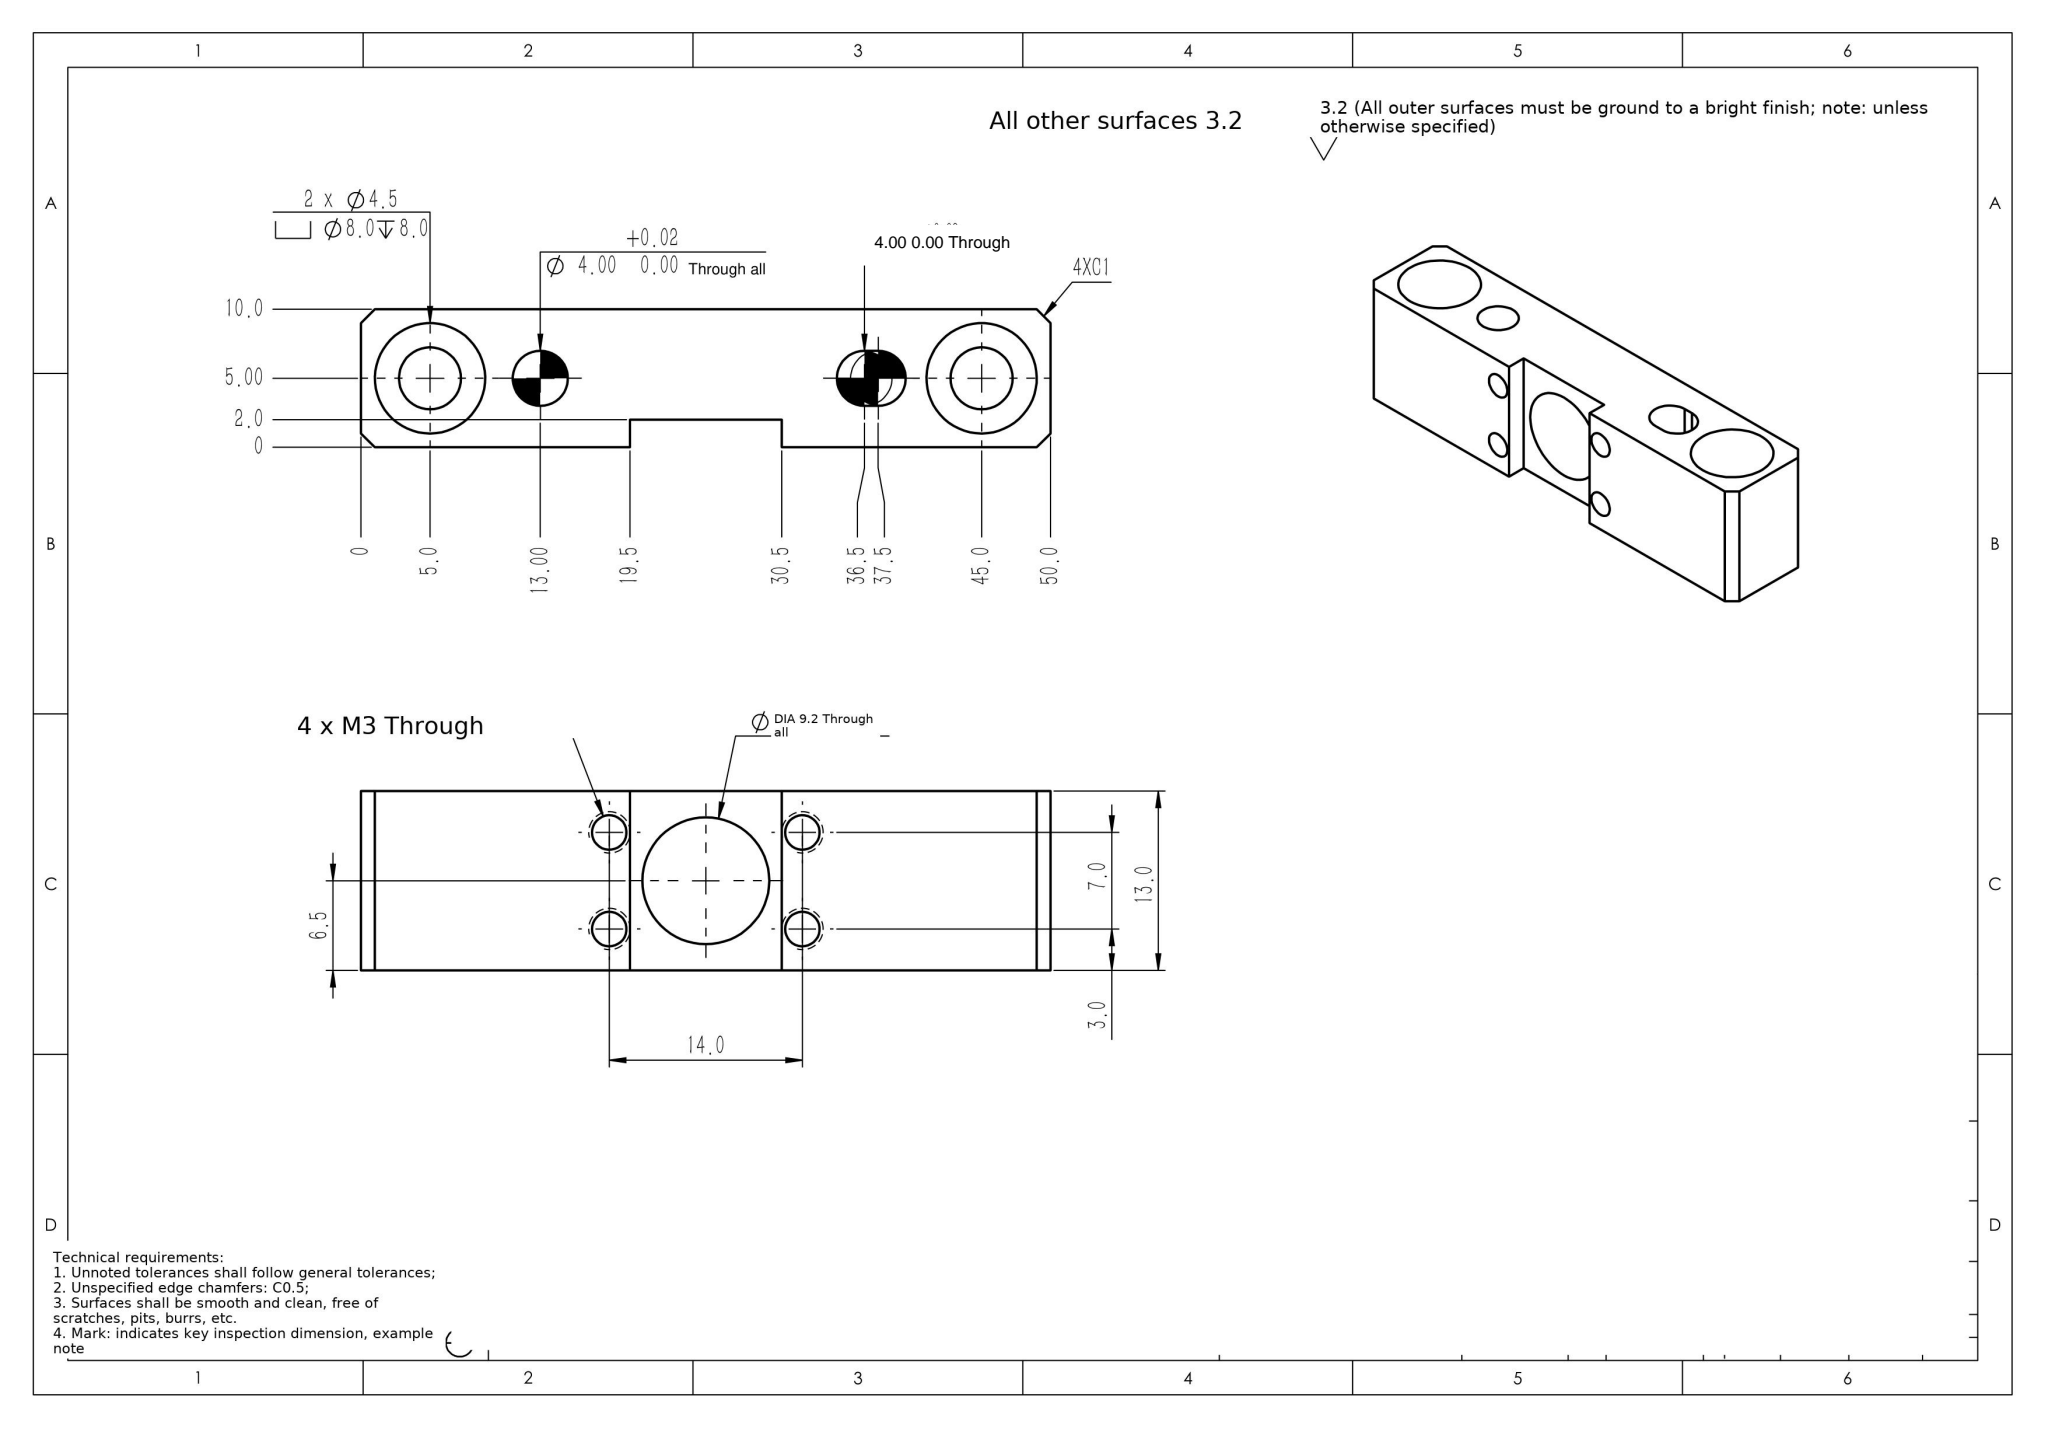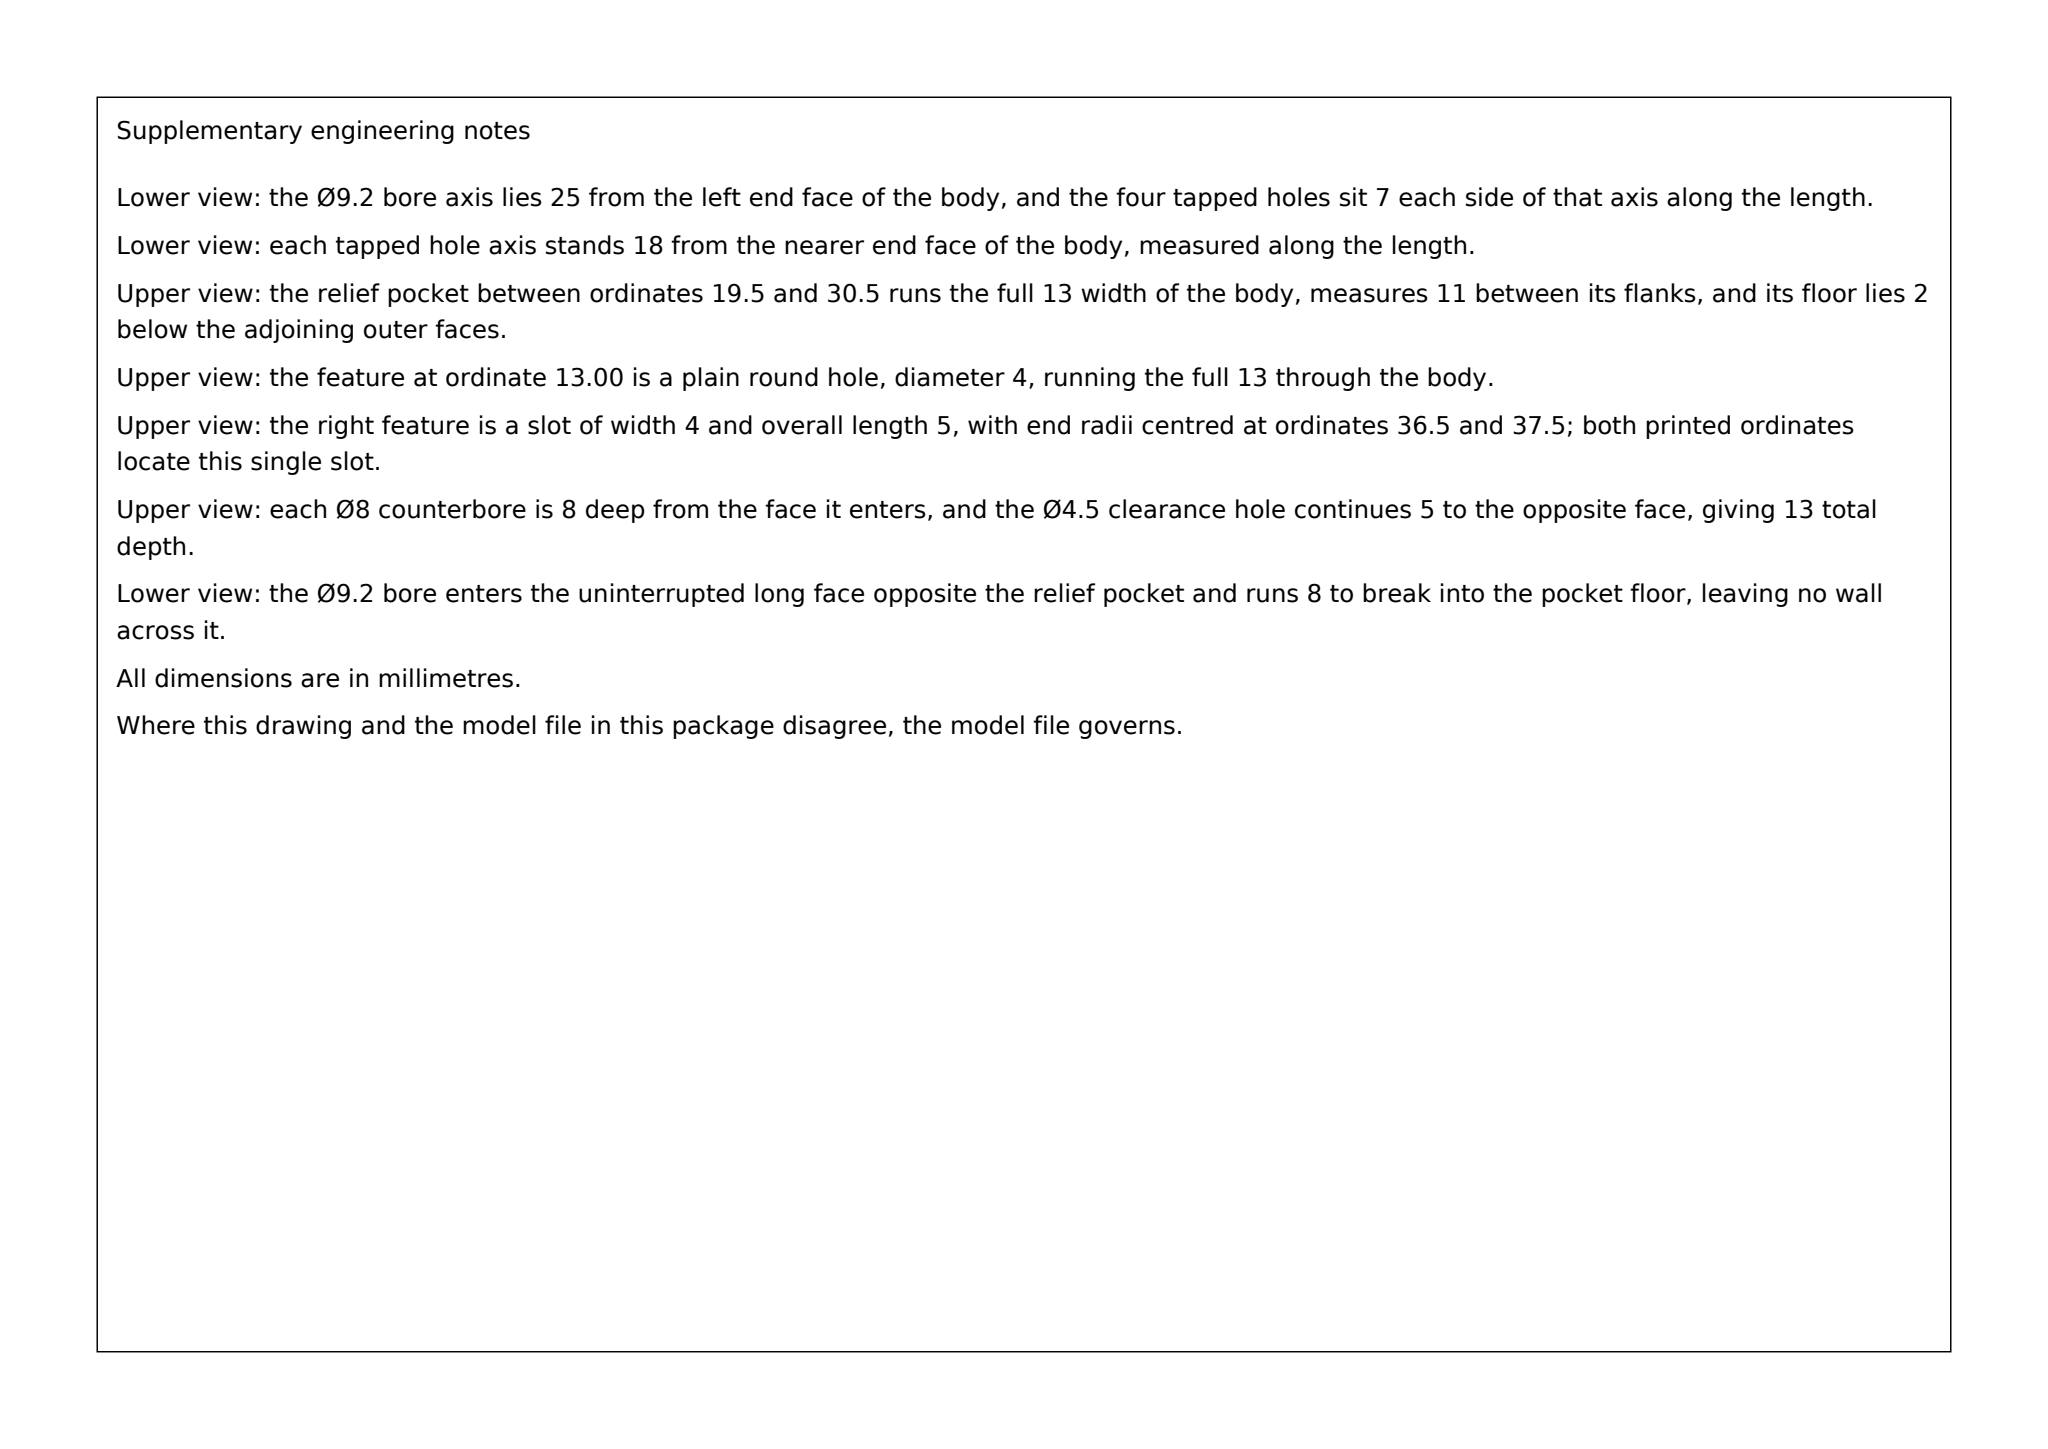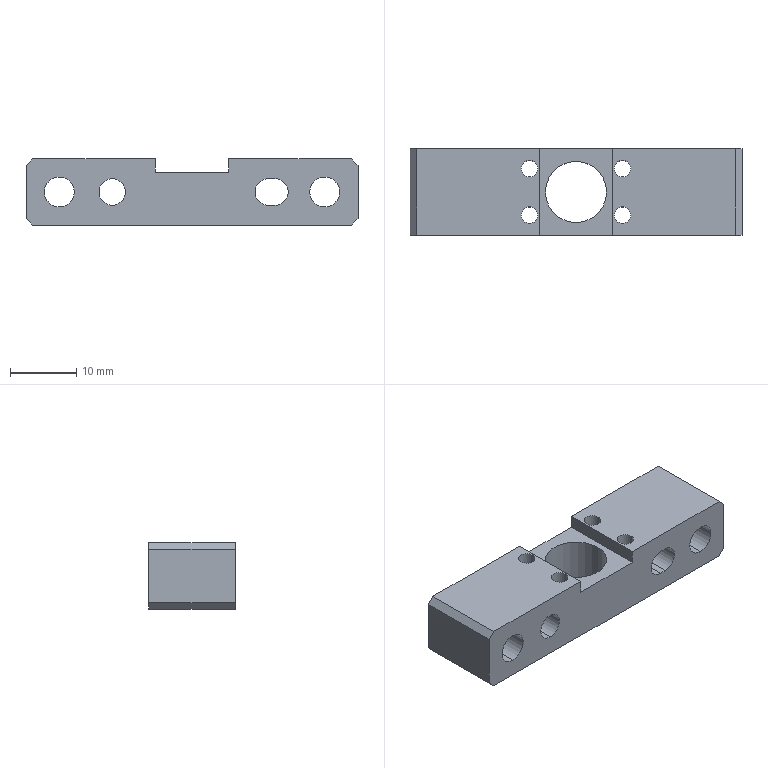Part | SolidWorks | mm | 1 solid | 40 faces | box 50 x 13 x 10 mm | volume 4118 mm3 | cylinder 22 | plane 18 | commonest cylinder face diameters 2.5 x8 4 x4 8 x4 4.5 x4 9.2 x2
Drawing notes:
CENTRAL STEP X19.5-X30.5: 2.0 DP x FULL 13.0 WIDTH THRU | from the solid: z planes 8.0 & 10.0 (2.0 step); x planes 19.5 & 30.5; y planes 0.0 & 13.0, no intermediate face
2X Ø4.5 THRU 13 WIDTH, C'BORE Ø8.0 DP 8.0 FROM Y13 FACE (FAR SIDE OF FRONT VIEW); CBORE FLOOR AT Y5.0, HOLE AXES AT X5.0 AND X45.0, Z5.0 | from the solid: cylinders dia4.5 axis y pos[5.0,null,5.0] & [45.0,null,5.0] len 5.0; dia8.0 axis y same positions len 8.0; axis_plane y=5.0 count 2 (counterbore floors) with bbox Y=13.0
2X Ø4.00 (+0.02/0) THRU FULL 13 WIDTH, AXES AT X36.5 AND X37.5, Z5.0 (OVERLAPPING SLOT-FORM HOLES) | from the solid: cylinders dia4.0 axis y pos[36.5,null,5.0] len 13.0 and pos[37.5,null,5.0] len 13.0
Ø9.2 THRU HOLE AXIS AT X25.0, Y6.5 FROM MIN-CORNER DATUM (KEY INSPECTION DIM) | from the solid: cylinder dia9.2 axis z pos[25.0,6.5,null] len 8.0
2X Ø4.5 THRU full 13.0 width, C'BORE Ø8.0 DP 8.0 MACHINED FROM THE Y=13.0 FACE (back face, opposite the Y0 datum face); C'BORE FLOOR AT Y=5.0 FROM Y0 FACE, Ø4.5 PORTION 5.0 LONG TO Y0 FACE; HOLE AXES AT X=5.0 AND X=45.0, Z=5.0 | from the solid: cylinders [4.5,"y",[5.0,null,5.0],5.0] and [4.5,"y",[45.0,null,5.0],5.0]; [8.0,"y",[5.0,null,5.0],8.0] and [8.0,"y",[45.0,null,5.0],8.0]; axis_planes ["y",5.0]:2 and ["y",13.0]:1
2X Ø4.00 THRU full 13.0 width (Y0 to Y13 faces), AXES AT X=36.5 AND X=37.5, Z=5.0 FROM BOTTOM | from the solid: cylinders [4.0,"y",[36.5,null,5.0],13.0] and [4.0,"y",[37.5,null,5.0],13.0]
Ø4.00 (+0.02/0) THRU FULL 13.0 WIDTH (Y0 TO Y13 FACES), HOLE AXIS AT X=13.0, Z=5.0 FROM MIN-CORNER DATUM | from the solid: cylinders[4.0,'y',[13.0,null,5.0],13.0] (count 2, coaxial through 13 mm width)
4X M3 THRU FULL 10.0 HEIGHT (Z0 TO Z10), AXES AT X=18.0 AND X=32.0 FROM X0 DATUM (14.0 APART, SYMMETRIC ABOUT X=25.0), Y=3.0 AND Y=10.0 FROM Y0 DATUM | from the solid: cylinders[2.5,'z',[18.0,3.0],10.0], [2.5,'z',[18.0,10.0],10.0], [2.5,'z',[32.0,3.0],10.0], [2.5,'z',[32.0,10.0],10.0]